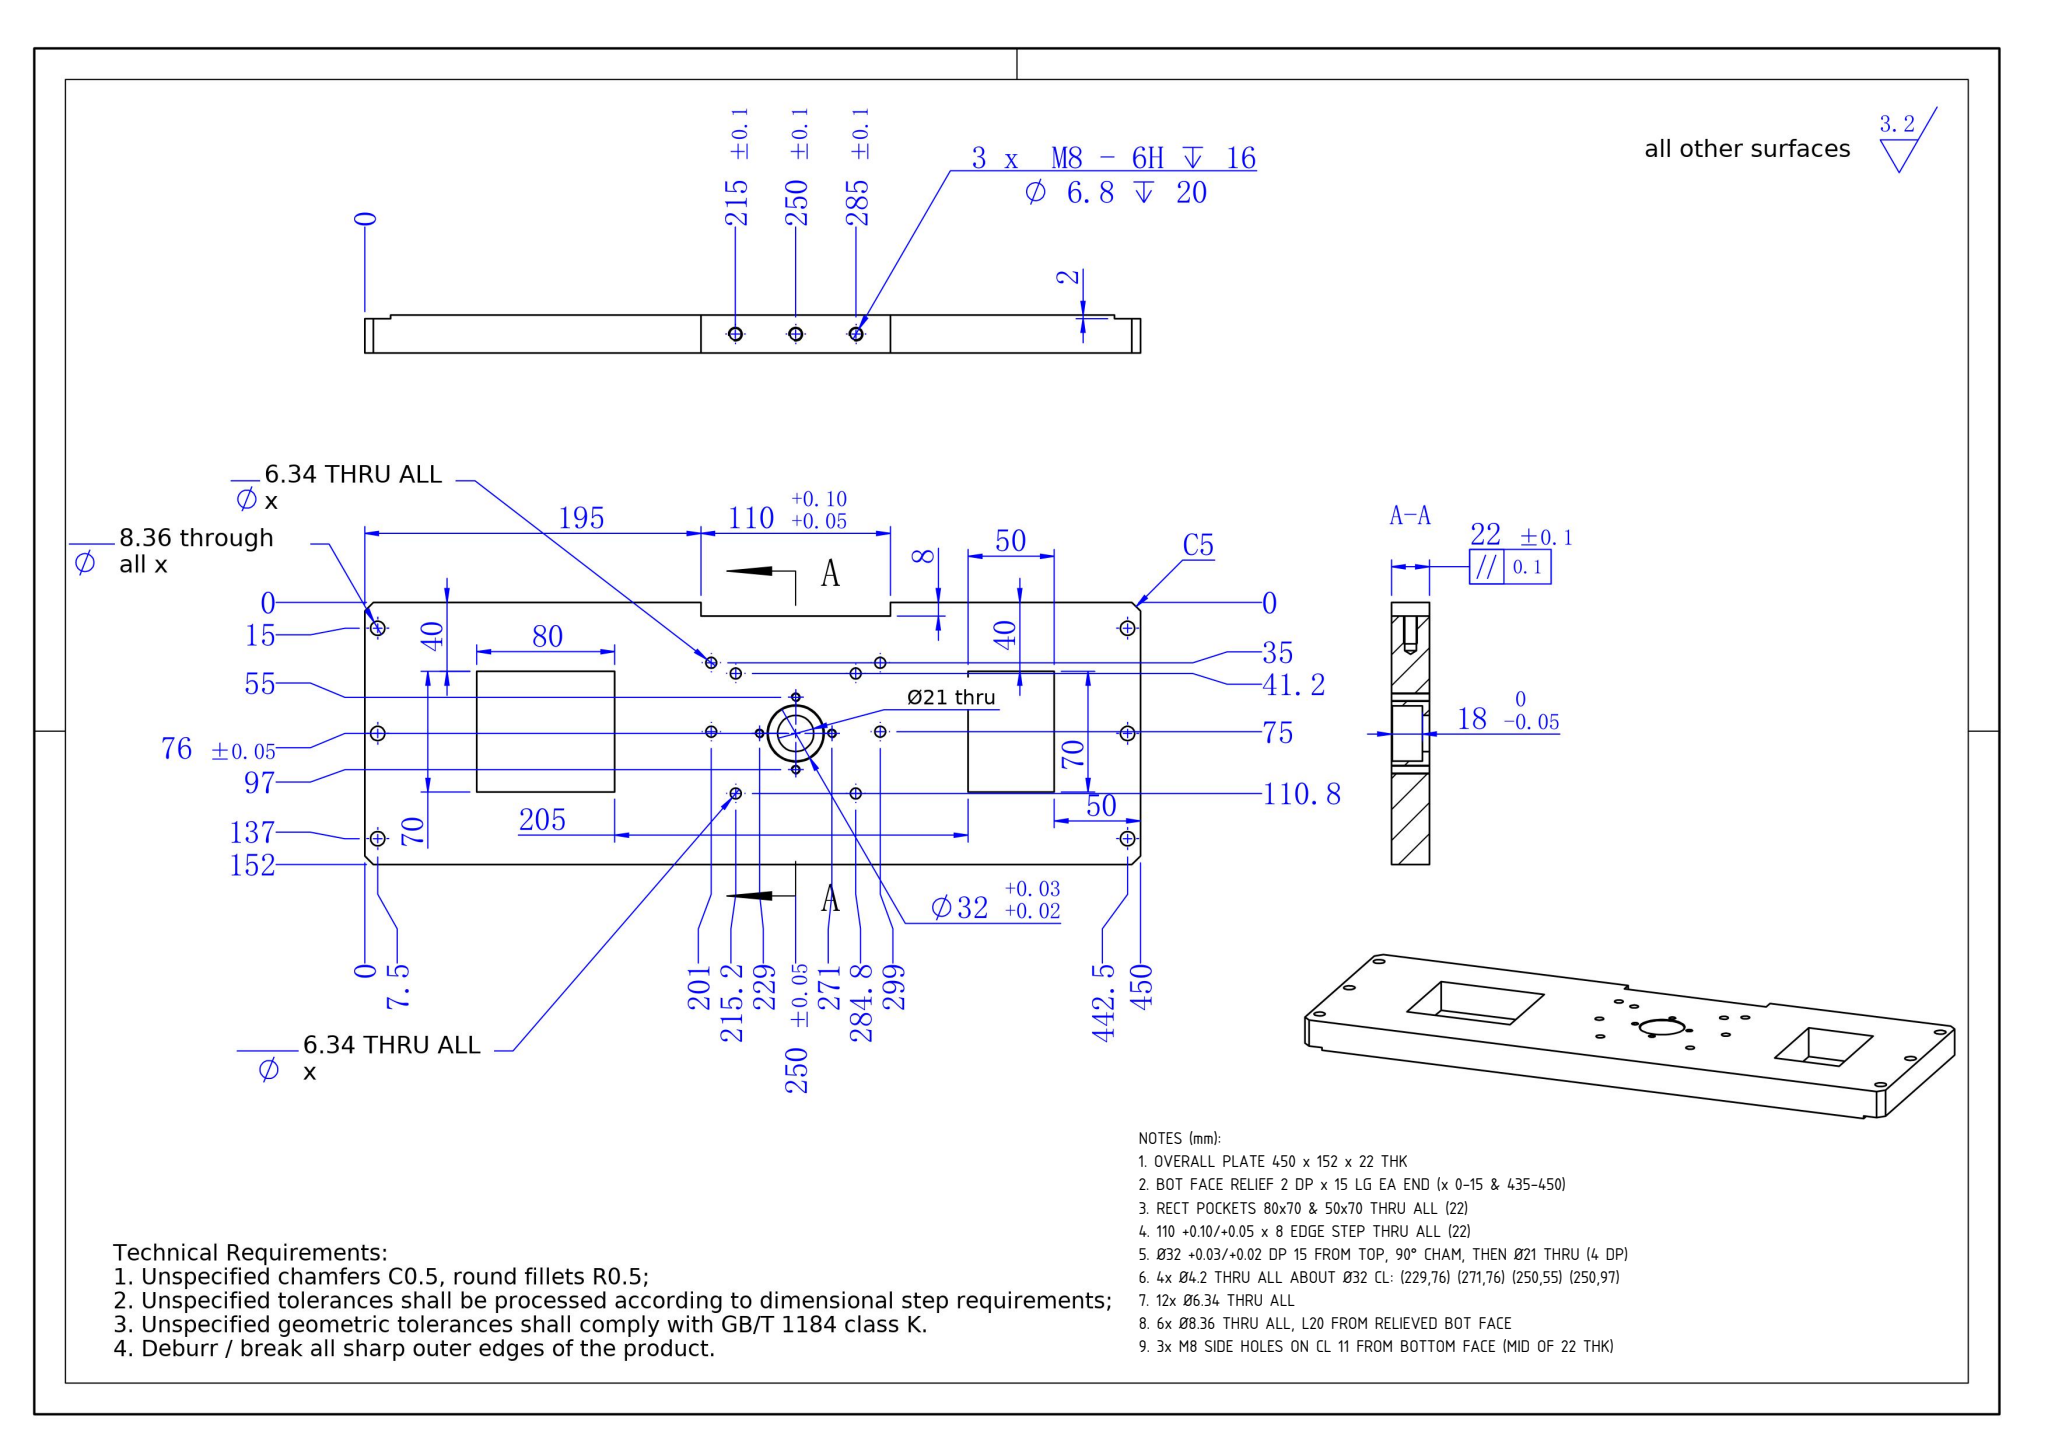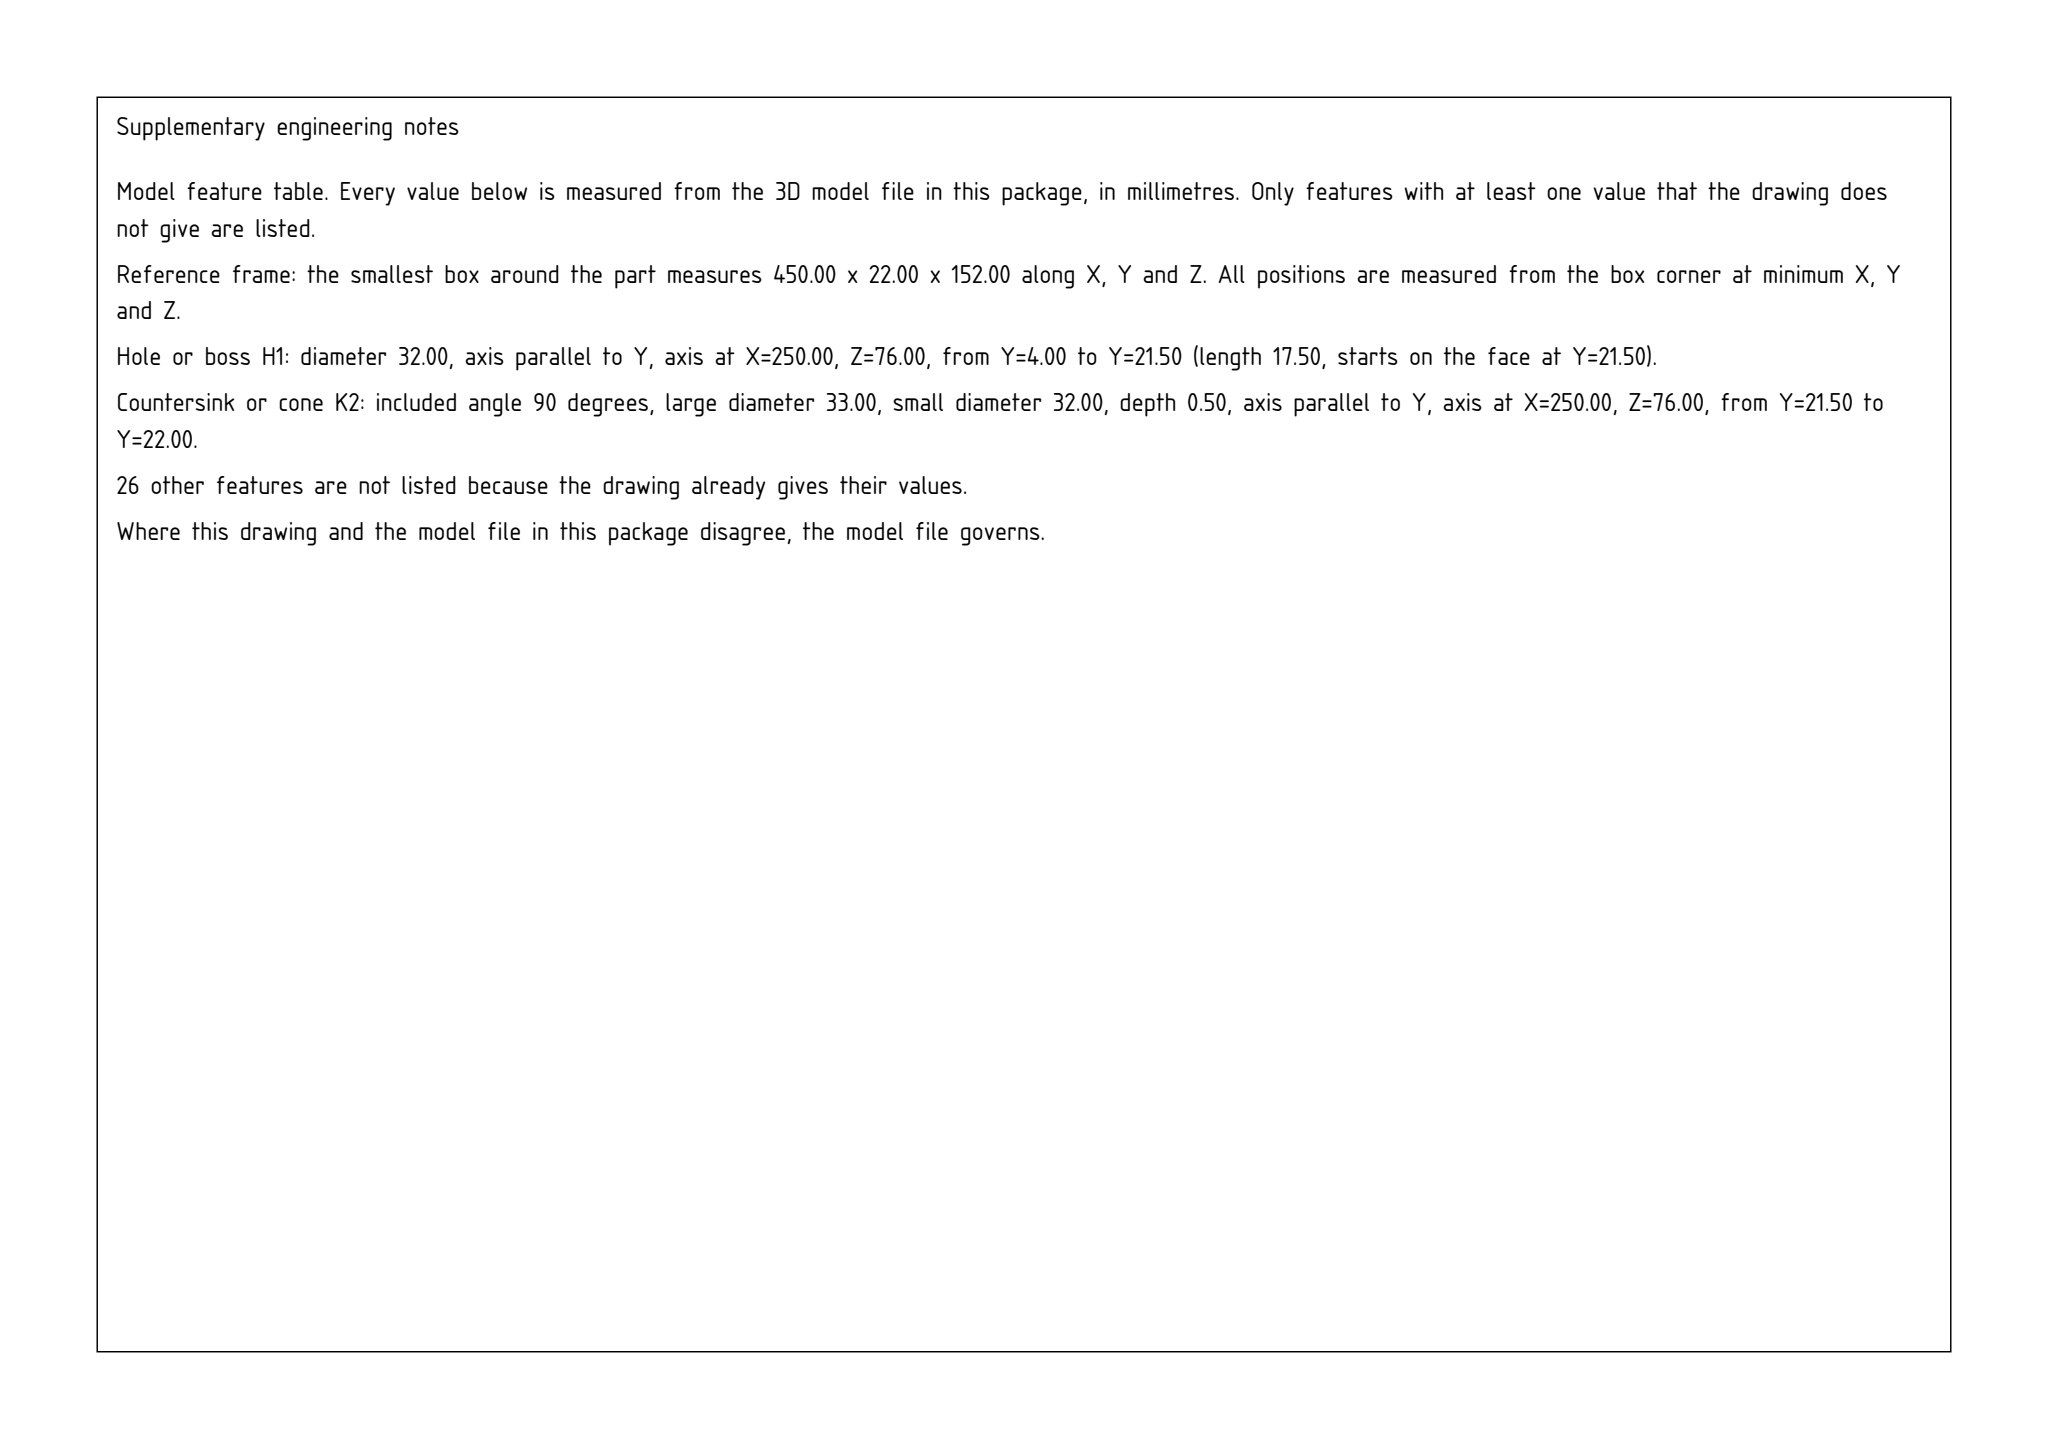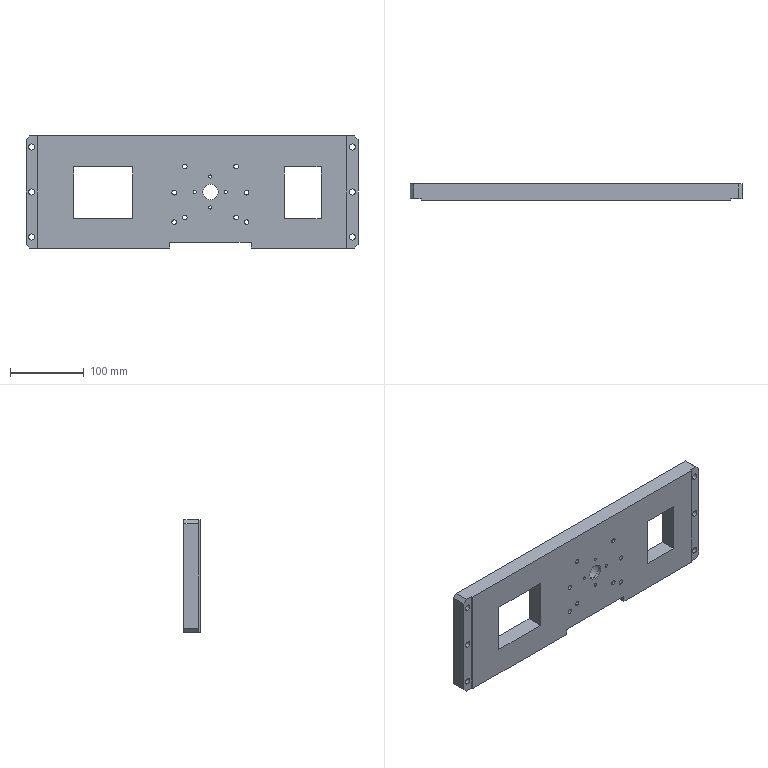Part | SolidWorks | mm | 1 solid | 81 faces | box 450 x 22 x 152 mm | volume 1243794 mm3 | cylinder 46 | plane 27 | cone 8 | commonest cylinder face diameters 6.3 x16 8.3 x12 4.2 x8 6.8 x6 21 x2 32 x2
Drawing notes:
OVERALL PLATE 450 x 152 x 22 THK | from the solid: bbox_xyz 450.0 x 22.0 x 152.0
BOT FACE RELIEF 2 DP x 15 LG EA END (x 0-15 & 435-450) | from the solid: y=2 planes (2 off) with x=15 and x=435 planes
RECT POCKETS 80x70 & 50x70 THRU ALL (22) | from the solid: Pocket walls x=65/145/350/400, z=40(2)/110(2); no y floor, so thru full 22 thk
110 +0.10/+0.05 x 8 EDGE STEP THRU ALL (22) | from the solid: x=195 & x=305 walls (110 wide), z=8 floor; no y plane bounding it
Ø32 +0.03/+0.02 DP 15 FROM TOP, 90° CHAM, THEN Ø21 THRU (4 DP) | from the solid: Cyl Ø32 L=17.5 + 90° cone ref Ø32 entry cham, flat at y=4; Ø21 L=4 from y=4 to y=0
4x Ø4.2 THRU ALL ABOUT Ø32 CL: (229,76) (271,76) (250,55) (250,97) | from the solid: cylinders dia 4.2, axis y, len 22 (full thk) at listed positions
12x Ø6.34 THRU ALL | from the solid: 12 Ø6.3 y-axis cylinders L=22 at x 201/215.2/284.8/299, z 35/41.2/75/110.8
6x Ø8.36 THRU ALL, L20 FROM RELIEVED BOT FACE | from the solid: 6 Ø8.3 y-axis cyls L=20 at x=7.5/442.5, z=15/76/137 (22 less 2 relief)
3x M8 SIDE HOLES ON CL 11 FROM BOTTOM FACE (MID OF 22 THK) | from the solid: cylinders dia 6.8 axis z at y=11.0, bbox y=22.0
build123d program:
from build123d import *

# Parameters (mm, degrees)
SKETCH1_W                  = 450
SKETCH1_H                  = 152
BOSS_EXTRUDE1_DEPTH        = 22
F_8_3_8_3_DIAMETER_SLOT1_D = 8.3
SKETCH4_R                  = 16
CUT_EXTRUDE1_DEPTH         = 18
SKETCH5_R                  = 10.5
CUT_EXTRUDE2_DEPTH         = 20
CHAMFER1_SIZE              = 5
F_6_3_6_3_DIAMETER_HOLE1_D = 6.3
CHAMFER2_SIZE              = 0.5
M5_TAPPED_HOLE1_D          = 4.2
SKETCH21_W                 = 110
SKETCH21_H                 = 22
CUT_EXTRUDE3_DEPTH         = 8
M8_TAPPED_HOLE1_D          = 6.8
M8_TAPPED_HOLE1_DEPTH      = 20
M8_TAPPED_HOLE1_TIP        = 2.043
F_6_3_6_3_DIAMETER_HOLE2_D = 6.3
SKETCH27_W                 = 15
SKETCH27_H                 = 2
CUT_EXTRUDE4_DEPTH         = 476.487
SKETCH28_W                 = 80
SKETCH28_H                 = 70
SKETCH28_W_2               = 50
CUT_EXTRUDE5_DEPTH         = 93


with BuildPart() as part:
    # Sketch1 → Boss-Extrude1 (new body)
    with BuildSketch(Plane(origin=(0, 0, 0), x_dir=(1, 0, 0), z_dir=(0, 1, 0))):
        with Locations((225, 76)):
            Rectangle(SKETCH1_W, SKETCH1_H)
    extrude(amount=BOSS_EXTRUDE1_DEPTH)

    # 8.3 _8.3_ Diameter Slot1 (through all)
    with Locations(Plane(origin=(0, 22, 0), x_dir=(1, 0, 0), z_dir=(0, 1, 0))):
        with Locations((7.5, 15), (442.5, 15), (7.5, 137), (442.5, 137), (7.5, 76), (442.5, 76)):
            Hole(F_8_3_8_3_DIAMETER_SLOT1_D / 2)

    # Sketch4 → Cut-Extrude1 (cut)
    with BuildSketch(Plane(origin=(0, 22, 0), x_dir=(1, 0, 0), z_dir=(0, 1, 0))):
        with Locations(Location((250, 76, 0), (0, 0, 270))):
            Circle(SKETCH4_R)
    extrude(amount=-CUT_EXTRUDE1_DEPTH, mode=Mode.SUBTRACT)

    # Sketch5 → Cut-Extrude2 (cut)
    with BuildSketch(Plane(origin=(0, 4, 0), x_dir=(1, 0, 0), z_dir=(0, 1, 0))):
        with Locations(Location((250, 76, 0), (0, 0, 270))):
            Circle(SKETCH5_R)
    extrude(amount=-CUT_EXTRUDE2_DEPTH, mode=Mode.SUBTRACT)

    # Chamfer1
    chamfer1_edges = [part.edges().sort_by_distance(p)[0] for p in [
        (0, 11, -152),
        (450, 11, -152),
        (450, 11, 0),
        (0, 11, 0),
    ]]
    chamfer(chamfer1_edges, length=CHAMFER1_SIZE)

    # 6.3 _6.3_ Diameter Hole1 (through all)
    with Locations(Plane(origin=(0, 22, 0), x_dir=(1, 0, 0), z_dir=(0, 1, 0))):
        with Locations((215.2, 110.8), (284.8, 110.8), (284.8, 41.2), (215.2, 41.2)):
            Hole(F_6_3_6_3_DIAMETER_HOLE1_D / 2)

    # Chamfer2
    chamfer2_edges = [part.edges().sort_by_distance(p)[0] for p in [
        (250, 22, -92),
    ]]
    chamfer(chamfer2_edges, length=CHAMFER2_SIZE)

    # M5 Tapped Hole1 (through all)
    with Locations(Plane(origin=(0, 22, 0), x_dir=(1, 0, 0), z_dir=(0, 1, 0))):
        with Locations((271, 76), (250, 55), (229, 76), (250, 97)):
            Hole(M5_TAPPED_HOLE1_D / 2)

    # Sketch21 → Cut-Extrude3 (cut)
    with BuildSketch(Plane(origin=(0, 0, -152), x_dir=(-1, 0, 0), z_dir=(0, 0, -1))):
        with Locations((-250, 11)):
            Rectangle(SKETCH21_W, SKETCH21_H)
    extrude(amount=-CUT_EXTRUDE3_DEPTH, mode=Mode.SUBTRACT)

    # M8 Tapped Hole1
    with Locations(Plane(origin=(0, 0, -144), x_dir=(-1, 0, 0), z_dir=(0, 0, -1))):
        with Locations((-215, 11), (-250, 11), (-285, 11)):
            Hole(M8_TAPPED_HOLE1_D / 2, depth=M8_TAPPED_HOLE1_DEPTH)
            with Locations((0, 0, -(M8_TAPPED_HOLE1_DEPTH + M8_TAPPED_HOLE1_TIP / 2))):  # 118° drill point
                Cone(0, M8_TAPPED_HOLE1_D / 2, M8_TAPPED_HOLE1_TIP, mode=Mode.SUBTRACT)

    # 6.3 _6.3_ Diameter Hole2 (through all)
    with Locations(Plane(origin=(0, 22, 0), x_dir=(1, 0, 0), z_dir=(0, 1, 0))):
        with Locations((201, 117), (201, 77)):
            f_6_3_6_3_diameter_hole2 = Hole(F_6_3_6_3_DIAMETER_HOLE2_D / 2)

    # Mirror1: 6.3 _6.3_ Diameter Hole2 across plane
    add(f_6_3_6_3_diameter_hole2.mirror(Plane.ZY.offset(-250)), mode=Mode.SUBTRACT)

    # Sketch27 → Cut-Extrude4 (cut, through all)
    with BuildSketch(Plane.XY):
        with Locations((442.5, 1)):
            Rectangle(SKETCH27_W, SKETCH27_H)
    cut_extrude4 = extrude(amount=-CUT_EXTRUDE4_DEPTH, mode=Mode.SUBTRACT)

    # Mirror3: Cut-Extrude4 across plane
    add(cut_extrude4.mirror(Plane.ZY.offset(-225)), mode=Mode.SUBTRACT)

    # Sketch28 → Cut-Extrude5 (cut)
    with BuildSketch(Plane(origin=(0, 22, 0), x_dir=(1, 0, 0), z_dir=(0, 1, 0))):
        with Locations((105, 77)):
            Rectangle(SKETCH28_W, SKETCH28_H)
        with Locations((375, 77)):
            Rectangle(SKETCH28_W_2, SKETCH28_H)
    extrude(amount=-CUT_EXTRUDE5_DEPTH, mode=Mode.SUBTRACT)


solid = part.part